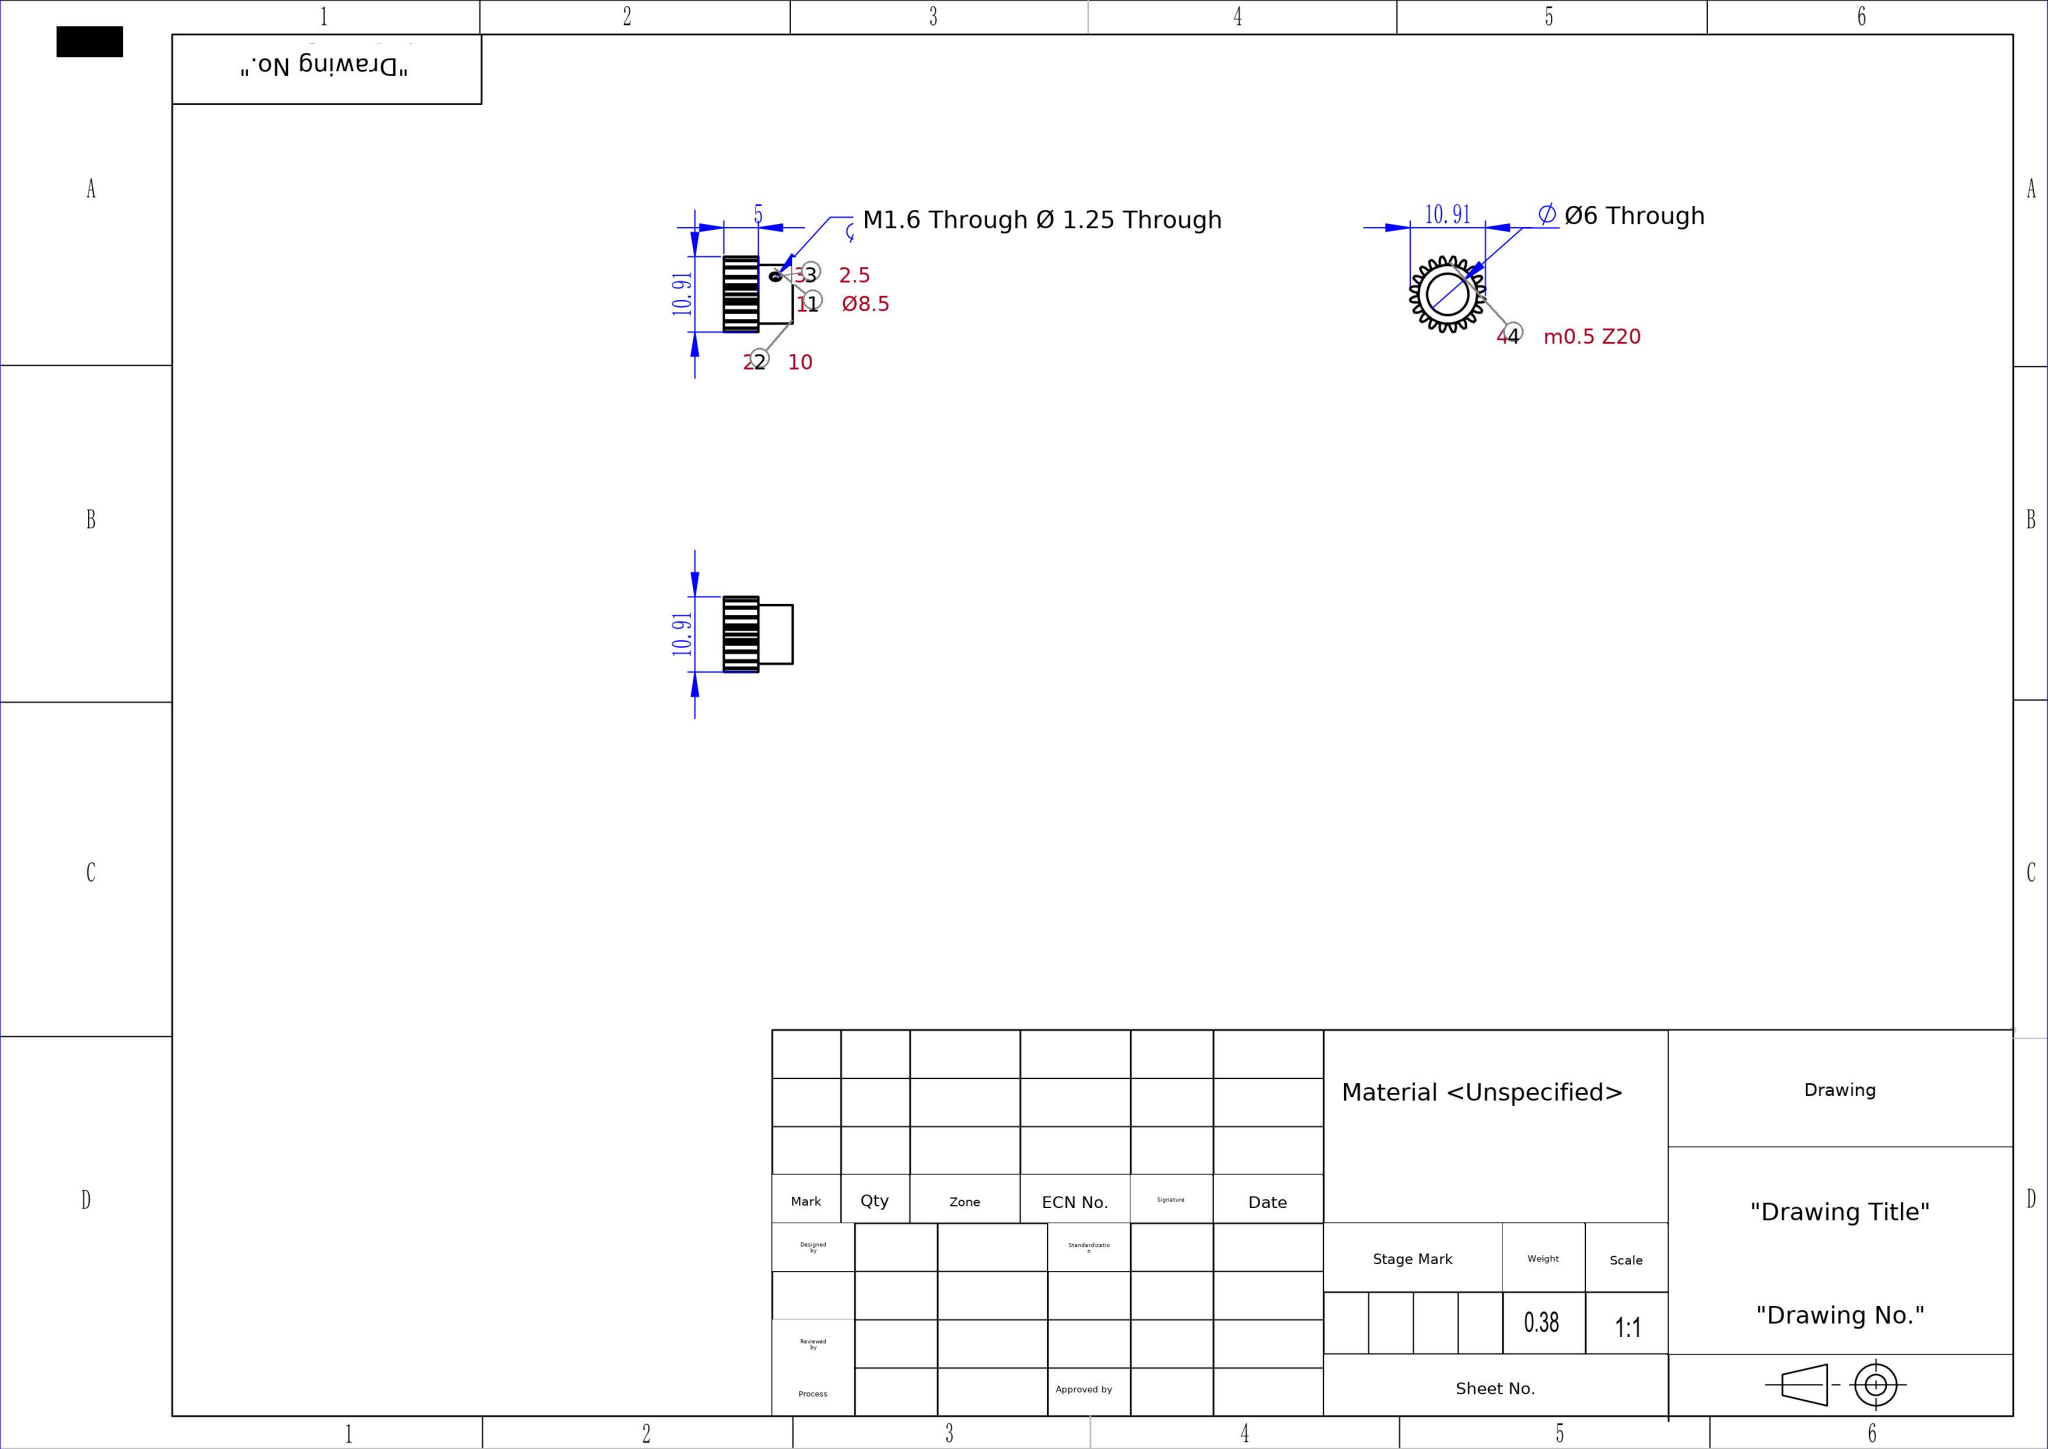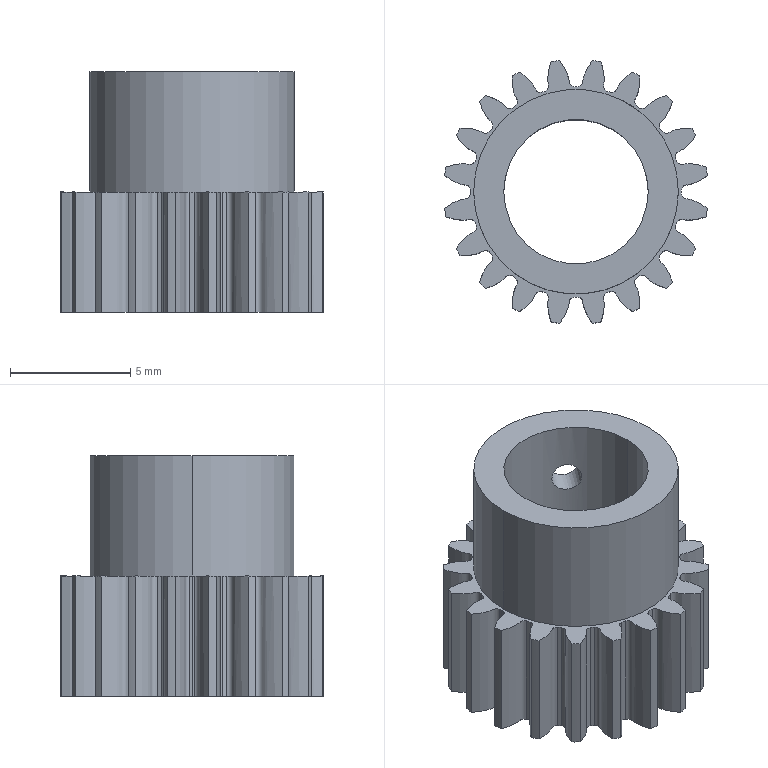Part | SolidWorks | mm | 1 solid | 92 faces | box 10.91 x 10.91 x 10 mm | volume 385 mm3 | cylinder 47 | spline 40 | plane 3 | cone 2 | commonest cylinder face diameters 8.75 x21 11 x20 1.25 x2 8.5 x2 6 x2